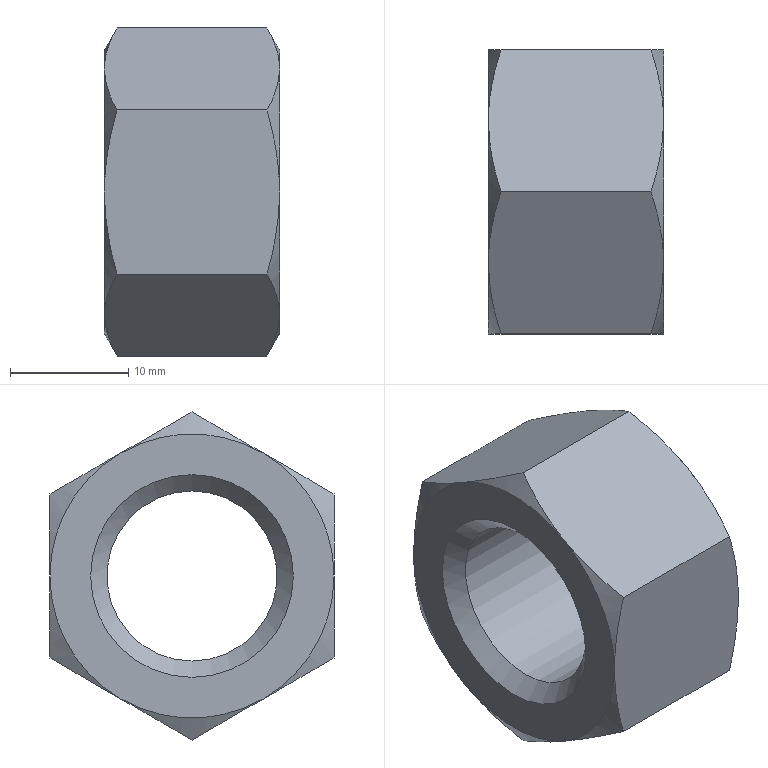Component | NX | GB-T6170_F-2000_M16X2 | 1 solid | 23 faces | volume 4858 mm3 | cone 14 | plane 8 | cylinder 1 | commonest cylinder face diameters 14.376 x1